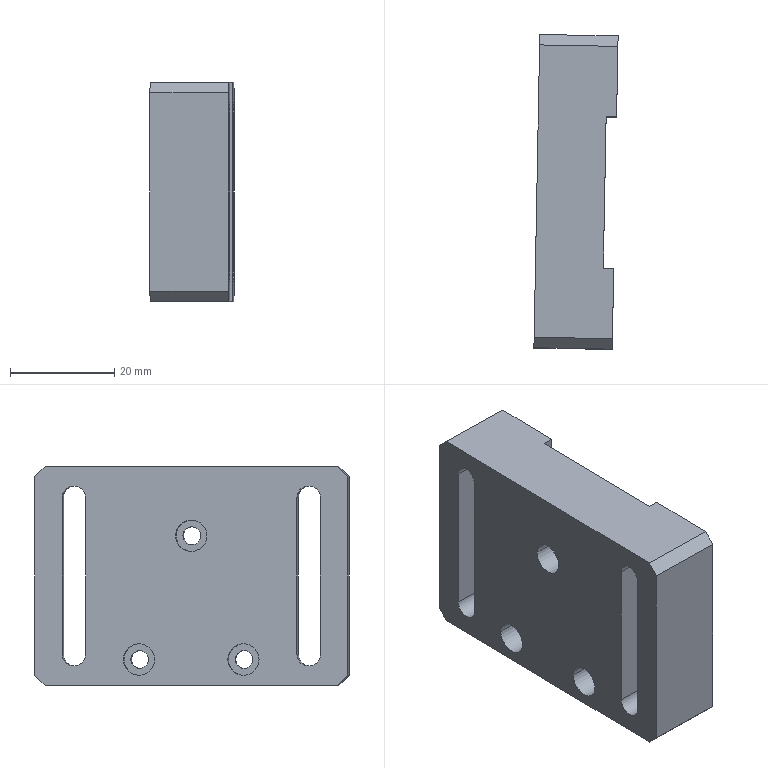Component | SolidWorks | DM17A08-04-008-1 | 1 solid | 37 faces | box 16.12 x 60.27 x 42 mm | volume 30017 mm3 | plane 21 | cylinder 16 | commonest cylinder face diameters 6 x6 3.4 x6 4.5 x4 | material 6061 Alloy
build123d program:
from build123d import *

# Parameters (mm, degrees)
SKETCH1_W                                            = 60
SKETCH1_H                                            = 42
BOSS_EXTRUDE1_DEPTH                                  = 15
SKETCH2_W                                            = 29
SKETCH2_H                                            = 42
CUT_EXTRUDE1_DEPTH                                   = 2
CHAMFER1_SIZE                                        = 2
HOLE_SIZE_ACCORDING_TO_TYPE_5_OF_HEXAGON_D           = 3.4
HOLE_SIZE_ACCORDING_TO_TYPE_5_OF_HEXAGON_CBORE_D     = 6
HOLE_SIZE_ACCORDING_TO_TYPE_5_OF_HEXAGON_CBORE_DEPTH = 6
CUT_EXTRUDE2_DEPTH                                   = 40.573


with BuildPart() as part:
    # Sketch1 → Boss-Extrude1 (new body)
    with BuildSketch(Plane.XY):
        Rectangle(SKETCH1_W, SKETCH1_H)
    extrude(amount=BOSS_EXTRUDE1_DEPTH)

    # Sketch2 → Cut-Extrude1 (cut)
    with BuildSketch(Plane.XY.offset(15)):
        Rectangle(SKETCH2_W, SKETCH2_H)
    extrude(amount=-CUT_EXTRUDE1_DEPTH, mode=Mode.SUBTRACT)

    # Chamfer1
    chamfer1_edges = [part.edges().sort_by_distance(p)[0] for p in [
        (30, -21, 7.5),
        (-30, -21, 7.5),
        (-30, 21, 7.5),
        (30, 21, 7.5),
    ]]
    chamfer(chamfer1_edges, length=CHAMFER1_SIZE)

    # Hole Size_According to_Type 5 of Hexagon (through all)
    with Locations(Plane(origin=(0, 0, 0), x_dir=(-1, 0, 0), z_dir=(0, 0, -1))):
        with Locations((0, 7.7), (-10, -16), (10, -16), (-49.439, -3.967)):
            CounterBoreHole(HOLE_SIZE_ACCORDING_TO_TYPE_5_OF_HEXAGON_D / 2, HOLE_SIZE_ACCORDING_TO_TYPE_5_OF_HEXAGON_CBORE_D / 2, HOLE_SIZE_ACCORDING_TO_TYPE_5_OF_HEXAGON_CBORE_DEPTH)

    # Sketch5 → Cut-Extrude2 (cut, through all)
    with BuildSketch(Plane.XY.offset(15)):
        with BuildLine():
            Line((-24.75, -15), (-24.75, 15))
            ThreePointArc((-24.75, 15), (-22.5, 17.25), (-20.25, 15))
            Line((-20.25, 15), (-20.25, -15))
            ThreePointArc((-20.25, -15), (-22.5, -17.25), (-24.75, -15))
        make_face()
        with BuildLine():
            Line((24.75, -15), (24.75, 15))
            ThreePointArc((24.75, 15), (22.5, 17.25), (20.25, 15))
            Line((20.25, 15), (20.25, -15))
            ThreePointArc((20.25, -15), (22.5, -17.25), (24.75, -15))
        make_face()
    extrude(amount=-CUT_EXTRUDE2_DEPTH, mode=Mode.SUBTRACT)


solid = part.part

# Placed as in the assembly
solid = solid.moved(Location((512.46, 339.783, 1046.565), (90, 88.927, 0)))